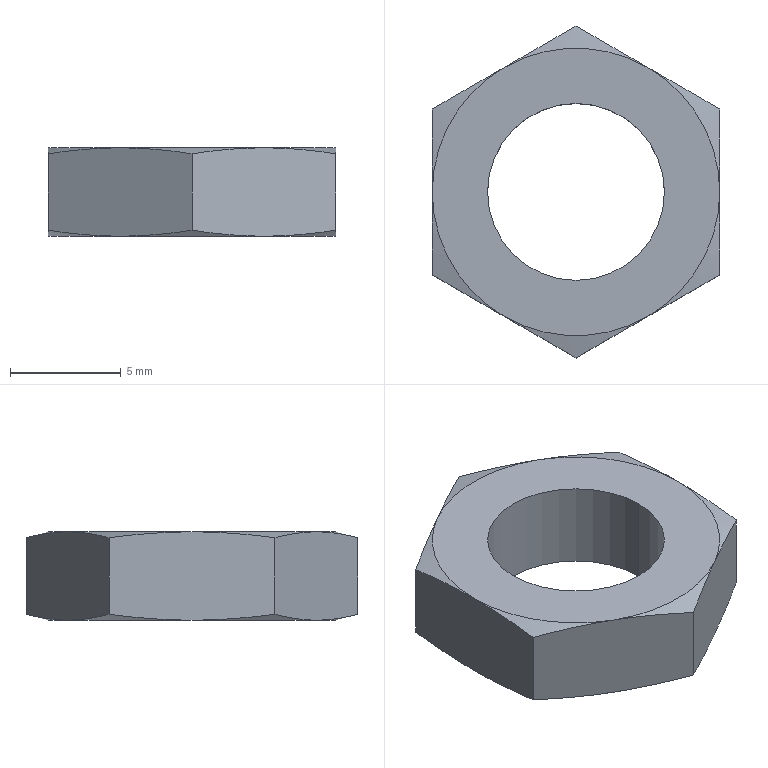Component | SolidWorks | GB_T6174-2000[HexThinNutNoChamferM8]-1 | 1 solid | 22 faces | box 13 x 15.01 x 4 mm | volume 382 mm3 | cone 12 | plane 8 | cylinder 2 | commonest cylinder face diameters 8 x2
build123d program:
from build123d import *

# Parameters (mm, degrees)
SKETCH1_R          = 4
BASE_EXTRUDE_DEPTH = 4
SKETCH2_OUTSIDE_W  = 106.414
SKETCH2_OUTSIDE_H  = 108.426
SKETCH2_OUTSIDE_R  = 6.5
CUT_EXTRUDE1_DEPTH = 11.704
CUT_EXTRUDE1_DRAFT = -75
SKETCH3_OUTSIDE_W  = 106.414
SKETCH3_OUTSIDE_H  = 108.426
SKETCH3_OUTSIDE_R  = 6.5
CUT_EXTRUDE2_DEPTH = 11.704
CUT_EXTRUDE2_DRAFT = -75


with BuildPart() as part:
    # Sketch1 → Base-Extrude (new body)
    with BuildSketch(Plane.XY):
        Polygon((0, 7.506), (-6.5, 3.753), (-6.5, -3.753), (0, -7.506), (6.5, -3.753), (6.5, 3.753), align=None)
        Circle(SKETCH1_R, mode=Mode.SUBTRACT)
    extrude(amount=BASE_EXTRUDE_DEPTH)


with BuildPart() as cut_extrude1_tool:
    # Sketch2 outside → Cut-Extrude1 (with draft: the straight prism first)
    with BuildSketch(Plane(origin=(0, 0, 0), x_dir=(-1, 0, 0), z_dir=(0, 0, -1))):
        Rectangle(SKETCH2_OUTSIDE_W, SKETCH2_OUTSIDE_H)
        Circle(SKETCH2_OUTSIDE_R, mode=Mode.SUBTRACT)
    extrude(amount=-CUT_EXTRUDE1_DEPTH)
    # Cut-Extrude1: the draft: its side faces are tilted about the plane it starts from
    cut_extrude1_sides = [cut_extrude1_tool.faces().sort_by_distance(p)[0] for p in [
        (0, -54.213, 5.852),
        (-53.207, 0, 5.852),
        (0, 54.213, 5.852),
        (53.207, 0, 5.852),
        (6.5, 0, 5.852),
    ]]
    draft(cut_extrude1_sides, Plane(origin=(0, 0, 0), x_dir=(-1, 0, 0), z_dir=(0, 0, -1)), CUT_EXTRUDE1_DRAFT)


with BuildPart() as part_1:
    add(part.part)

    # Cut-Extrude1: cut by cut_extrude1_tool
    add(cut_extrude1_tool.part, mode=Mode.SUBTRACT)


with BuildPart() as cut_extrude2_tool:
    # Sketch3 outside → Cut-Extrude2 (with draft: the straight prism first)
    with BuildSketch(Plane.XY.offset(4)):
        Rectangle(SKETCH3_OUTSIDE_W, SKETCH3_OUTSIDE_H)
        Circle(SKETCH3_OUTSIDE_R, mode=Mode.SUBTRACT)
    extrude(amount=-CUT_EXTRUDE2_DEPTH)
    # Cut-Extrude2: the draft: its side faces are tilted about the plane it starts from
    cut_extrude2_sides = [cut_extrude2_tool.faces().sort_by_distance(p)[0] for p in [
        (0, -54.213, -1.852),
        (53.207, 0, -1.852),
        (0, 54.213, -1.852),
        (-53.207, 0, -1.852),
        (-6.5, 0, -1.852),
    ]]
    draft(cut_extrude2_sides, Plane.XY.offset(4), CUT_EXTRUDE2_DRAFT)


with BuildPart() as part_2:
    add(part_1.part)

    # Cut-Extrude2: cut by cut_extrude2_tool
    add(cut_extrude2_tool.part, mode=Mode.SUBTRACT)


solid = part_2.part

# Placed as in the assembly
solid = solid.moved(Location((483.792, -540.614, 1168.971), (0, 0, 0)))
STEP:
#1=COLOUR_RGB('',0.7922,0.8196,0.9333);
#2=FILL_AREA_STYLE_COLOUR('',#1);
#3=FILL_AREA_STYLE('',(#2));
#4=SURFACE_STYLE_FILL_AREA(#3);
#5=SURFACE_SIDE_STYLE('',(#4));
#6=SURFACE_STYLE_USAGE(.BOTH.,#5);
#7=PRESENTATION_STYLE_ASSIGNMENT((#6));
#8=CARTESIAN_POINT('',(18.889,-21.284,46.18));
#9=VERTEX_POINT('',#8);
#10=CARTESIAN_POINT('',(19.204,-21.284,46.18));
#11=VERTEX_POINT('',#10);
#12=CARTESIAN_POINT('',(19.047,-21.284,46.18));
#13=DIRECTION('',(0.,0.,1.));
#14=DIRECTION('',(1.,0.,0.));
#15=AXIS2_PLACEMENT_3D('',#12,#13,#14);
#16=CIRCLE('',#15,0.1575);
#17=EDGE_CURVE('',#9,#11,#16,.T.);
#18=ORIENTED_EDGE('',*,*,#17,.T.);
#19=CARTESIAN_POINT('',(19.204,-21.284,46.022));
#20=VERTEX_POINT('',#19);
#21=CARTESIAN_POINT('',(19.204,-21.284,46.18));
#22=DIRECTION('',(0.,0.,-1.));
#23=VECTOR('',#22,39.37);
#24=LINE('',#21,#23);
#25=EDGE_CURVE('',#11,#20,#24,.T.);
#26=ORIENTED_EDGE('',*,*,#25,.T.);
#27=CARTESIAN_POINT('',(18.889,-21.284,46.022));
#28=VERTEX_POINT('',#27);
#29=CARTESIAN_POINT('',(19.047,-21.284,46.022));
#30=DIRECTION('',(0.,0.,1.));
#31=DIRECTION('',(1.,0.,0.));
#32=AXIS2_PLACEMENT_3D('',#29,#30,#31);
#33=CIRCLE('',#32,0.1575);
#34=EDGE_CURVE('',#28,#20,#33,.T.);
#35=ORIENTED_EDGE('',*,*,#34,.F.);
#36=CARTESIAN_POINT('',(18.889,-21.284,46.18));
#37=DIRECTION('',(0.,0.,-1.));
#38=VECTOR('',#37,39.37);
#39=LINE('',#36,#38);
#40=EDGE_CURVE('',#9,#28,#39,.T.);
#41=ORIENTED_EDGE('',*,*,#40,.F.);
#42=EDGE_LOOP('',(#18,#26,#35,#41));
#43=FACE_OUTER_BOUND('',#42,.T.);
#44=CARTESIAN_POINT('',(19.047,-21.284,46.18));
#45=DIRECTION('',(0.,0.,-1.));
#46=DIRECTION('',(-1.,0.,0.));
#47=AXIS2_PLACEMENT_3D('',#44,#45,#46);
#48=CYLINDRICAL_SURFACE('',#47,0.1575);
#49=ADVANCED_FACE('',(#43),#48,.F.);
#50=CARTESIAN_POINT('',(19.303,-21.136,46.169));
#51=VERTEX_POINT('',#50);
#52=CARTESIAN_POINT('',(19.175,-21.062,46.18));
#53=VERTEX_POINT('',#52);
#54=CARTESIAN_POINT('',(19.303,-21.136,46.169));
#55=CARTESIAN_POINT('',(19.26,-21.112,46.176));
#56=CARTESIAN_POINT('',(19.218,-21.087,46.18));
#57=CARTESIAN_POINT('',(19.175,-21.062,46.18));
#58=B_SPLINE_CURVE_WITH_KNOTS('',3,(#54,#55,#56,#57),.UNSPECIFIED.,.F.,.F.,(4,4),(0.00000023,0.003753),.UNSPECIFIED.);
#59=EDGE_CURVE('',#51,#53,#58,.T.);
#60=ORIENTED_EDGE('',*,*,#59,.F.);
#61=CARTESIAN_POINT('',(19.303,-21.136,46.033));
#62=VERTEX_POINT('',#61);
#63=CARTESIAN_POINT('',(19.303,-21.136,46.18));
#64=DIRECTION('',(0.,0.,-1.));
#65=VECTOR('',#64,39.37);
#66=LINE('',#63,#65);
#67=EDGE_CURVE('',#51,#62,#66,.T.);
#68=ORIENTED_EDGE('',*,*,#67,.T.);
#69=CARTESIAN_POINT('',(19.175,-21.062,46.022));
#70=VERTEX_POINT('',#69);
#71=CARTESIAN_POINT('',(19.175,-21.062,46.022));
#72=CARTESIAN_POINT('',(19.218,-21.087,46.022));
#73=CARTESIAN_POINT('',(19.26,-21.112,46.026));
#74=CARTESIAN_POINT('',(19.303,-21.136,46.033));
#75=B_SPLINE_CURVE_WITH_KNOTS('',3,(#71,#72,#73,#74),.UNSPECIFIED.,.F.,.F.,(4,4),(0.003753,0.007506),.UNSPECIFIED.);
#76=EDGE_CURVE('',#70,#62,#75,.T.);
#77=ORIENTED_EDGE('',*,*,#76,.F.);
#78=CARTESIAN_POINT('',(19.047,-20.989,46.033));
#79=VERTEX_POINT('',#78);
#80=CARTESIAN_POINT('',(19.047,-20.989,46.033));
#81=CARTESIAN_POINT('',(19.09,-21.013,46.026));
#82=CARTESIAN_POINT('',(19.132,-21.038,46.022));
#83=CARTESIAN_POINT('',(19.175,-21.062,46.022));
#84=B_SPLINE_CURVE_WITH_KNOTS('',3,(#80,#81,#82,#83),.UNSPECIFIED.,.F.,.F.,(4,4),(0.00000023,0.003753),.UNSPECIFIED.);
#85=EDGE_CURVE('',#79,#70,#84,.T.);
#86=ORIENTED_EDGE('',*,*,#85,.F.);
#87=CARTESIAN_POINT('',(19.047,-20.989,46.169));
#88=VERTEX_POINT('',#87);
#89=CARTESIAN_POINT('',(19.047,-20.989,46.18));
#90=DIRECTION('',(0.,0.,-1.));
#91=VECTOR('',#90,39.37);
#92=LINE('',#89,#91);
#93=EDGE_CURVE('',#88,#79,#92,.T.);
#94=ORIENTED_EDGE('',*,*,#93,.F.);
#95=CARTESIAN_POINT('',(19.175,-21.062,46.18));
#96=CARTESIAN_POINT('',(19.132,-21.038,46.18));
#97=CARTESIAN_POINT('',(19.09,-21.013,46.176));
#98=CARTESIAN_POINT('',(19.047,-20.989,46.169));
#99=B_SPLINE_CURVE_WITH_KNOTS('',3,(#95,#96,#97,#98),.UNSPECIFIED.,.F.,.F.,(4,4),(0.003753,0.007506),.UNSPECIFIED.);
#100=EDGE_CURVE('',#53,#88,#99,.T.);
#101=ORIENTED_EDGE('',*,*,#100,.F.);
#102=EDGE_LOOP('',(#60,#68,#77,#86,#94,#101));
#103=FACE_OUTER_BOUND('',#102,.T.);
#104=CARTESIAN_POINT('',(19.303,-21.136,46.18));
#105=DIRECTION('',(-0.5,-0.866,0.));
#106=DIRECTION('',(0.866,-0.5,0.));
#107=AXIS2_PLACEMENT_3D('',#104,#105,#106);
#108=PLANE('',#107);
#109=ADVANCED_FACE('',(#103),#108,.F.);
#110=CARTESIAN_POINT('',(18.919,-21.062,46.18));
#111=VERTEX_POINT('',#110);
#112=CARTESIAN_POINT('',(19.047,-20.989,46.169));
#113=CARTESIAN_POINT('',(19.004,-21.013,46.176));
#114=CARTESIAN_POINT('',(18.962,-21.038,46.18));
#115=CARTESIAN_POINT('',(18.919,-21.062,46.18));
#116=B_SPLINE_CURVE_WITH_KNOTS('',3,(#112,#113,#114,#115),.UNSPECIFIED.,.F.,.F.,(4,4),(0.00000023,0.003753),.UNSPECIFIED.);
#117=EDGE_CURVE('',#88,#111,#116,.T.);
#118=ORIENTED_EDGE('',*,*,#117,.F.);
#119=ORIENTED_EDGE('',*,*,#93,.T.);
#120=CARTESIAN_POINT('',(18.919,-21.062,46.022));
#121=VERTEX_POINT('',#120);
#122=CARTESIAN_POINT('',(18.919,-21.062,46.022));
#123=CARTESIAN_POINT('',(18.962,-21.038,46.022));
#124=CARTESIAN_POINT('',(19.004,-21.013,46.026));
#125=CARTESIAN_POINT('',(19.047,-20.989,46.033));
#126=B_SPLINE_CURVE_WITH_KNOTS('',3,(#122,#123,#124,#125),.UNSPECIFIED.,.F.,.F.,(4,4),(0.003753,0.007506),.UNSPECIFIED.);
#127=EDGE_CURVE('',#121,#79,#126,.T.);
#128=ORIENTED_EDGE('',*,*,#127,.F.);
#129=CARTESIAN_POINT('',(18.791,-21.136,46.033));
#130=VERTEX_POINT('',#129);
#131=CARTESIAN_POINT('',(18.791,-21.136,46.033));
#132=CARTESIAN_POINT('',(18.834,-21.112,46.026));
#133=CARTESIAN_POINT('',(18.876,-21.087,46.022));
#134=CARTESIAN_POINT('',(18.919,-21.062,46.022));
#135=B_SPLINE_CURVE_WITH_KNOTS('',3,(#131,#132,#133,#134),.UNSPECIFIED.,.F.,.F.,(4,4),(0.00000023,0.003753),.UNSPECIFIED.);
#136=EDGE_CURVE('',#130,#121,#135,.T.);
#137=ORIENTED_EDGE('',*,*,#136,.F.);
#138=CARTESIAN_POINT('',(18.791,-21.136,46.169));
#139=VERTEX_POINT('',#138);
#140=CARTESIAN_POINT('',(18.791,-21.136,46.18));
#141=DIRECTION('',(0.,0.,-1.));
#142=VECTOR('',#141,39.37);
#143=LINE('',#140,#142);
#144=EDGE_CURVE('',#139,#130,#143,.T.);
#145=ORIENTED_EDGE('',*,*,#144,.F.);
#146=CARTESIAN_POINT('',(18.919,-21.062,46.18));
#147=CARTESIAN_POINT('',(18.876,-21.087,46.18));
#148=CARTESIAN_POINT('',(18.834,-21.112,46.176));
#149=CARTESIAN_POINT('',(18.791,-21.136,46.169));
#150=B_SPLINE_CURVE_WITH_KNOTS('',3,(#146,#147,#148,#149),.UNSPECIFIED.,.F.,.F.,(4,4),(0.003753,0.007506),.UNSPECIFIED.);
#151=EDGE_CURVE('',#111,#139,#150,.T.);
#152=ORIENTED_EDGE('',*,*,#151,.F.);
#153=EDGE_LOOP('',(#118,#119,#128,#137,#145,#152));
#154=FACE_OUTER_BOUND('',#153,.T.);
#155=CARTESIAN_POINT('',(19.047,-20.989,46.18));
#156=DIRECTION('',(0.5,-0.866,0.));
#157=DIRECTION('',(0.866,0.5,0.));
#158=AXIS2_PLACEMENT_3D('',#155,#156,#157);
#159=PLANE('',#158);
#160=ADVANCED_FACE('',(#154),#159,.F.);
#161=CARTESIAN_POINT('',(18.791,-21.284,46.18));
#162=VERTEX_POINT('',#161);
#163=CARTESIAN_POINT('',(18.791,-21.136,46.169));
#164=CARTESIAN_POINT('',(18.791,-21.185,46.176));
#165=CARTESIAN_POINT('',(18.791,-21.235,46.18));
#166=CARTESIAN_POINT('',(18.791,-21.284,46.18));
#167=B_SPLINE_CURVE_WITH_KNOTS('',3,(#163,#164,#165,#166),.UNSPECIFIED.,.F.,.F.,(4,4),(0.01751,0.02129),.UNSPECIFIED.);
#168=EDGE_CURVE('',#139,#162,#167,.T.);
#169=ORIENTED_EDGE('',*,*,#168,.F.);
#170=ORIENTED_EDGE('',*,*,#144,.T.);
#171=CARTESIAN_POINT('',(18.791,-21.284,46.022));
#172=VERTEX_POINT('',#171);
#173=CARTESIAN_POINT('',(18.791,-21.284,46.022));
#174=CARTESIAN_POINT('',(18.791,-21.235,46.022));
#175=CARTESIAN_POINT('',(18.791,-21.185,46.027));
#176=CARTESIAN_POINT('',(18.791,-21.136,46.033));
#177=B_SPLINE_CURVE_WITH_KNOTS('',3,(#173,#174,#175,#176),.UNSPECIFIED.,.F.,.F.,(4,4),(0.01018,0.01396),.UNSPECIFIED.);
#178=EDGE_CURVE('',#172,#130,#177,.T.);
#179=ORIENTED_EDGE('',*,*,#178,.F.);
#180=CARTESIAN_POINT('',(18.791,-21.432,46.033));
#181=VERTEX_POINT('',#180);
#182=CARTESIAN_POINT('',(18.791,-21.432,46.033));
#183=CARTESIAN_POINT('',(18.791,-21.407,46.03));
#184=CARTESIAN_POINT('',(18.791,-21.383,46.027));
#185=CARTESIAN_POINT('',(18.791,-21.333,46.023));
#186=CARTESIAN_POINT('',(18.791,-21.309,46.022));
#187=CARTESIAN_POINT('',(18.791,-21.284,46.022));
#188=B_SPLINE_CURVE_WITH_KNOTS('',3,(#182,#183,#184,#185,#186,#187),.UNSPECIFIED.,.F.,.F.,(4,2,4),(0.006406,0.008292,0.01018),.UNSPECIFIED.);
#189=EDGE_CURVE('',#181,#172,#188,.T.);
#190=ORIENTED_EDGE('',*,*,#189,.F.);
#191=CARTESIAN_POINT('',(18.791,-21.432,46.169));
#192=VERTEX_POINT('',#191);
#193=CARTESIAN_POINT('',(18.791,-21.432,46.18));
#194=DIRECTION('',(0.,0.,-1.));
#195=VECTOR('',#194,39.37);
#196=LINE('',#193,#195);
#197=EDGE_CURVE('',#192,#181,#196,.T.);
#198=ORIENTED_EDGE('',*,*,#197,.F.);
#199=CARTESIAN_POINT('',(18.791,-21.284,46.18));
#200=CARTESIAN_POINT('',(18.791,-21.309,46.18));
#201=CARTESIAN_POINT('',(18.791,-21.333,46.179));
#202=CARTESIAN_POINT('',(18.791,-21.383,46.175));
#203=CARTESIAN_POINT('',(18.791,-21.407,46.173));
#204=CARTESIAN_POINT('',(18.791,-21.432,46.169));
#205=B_SPLINE_CURVE_WITH_KNOTS('',3,(#199,#200,#201,#202,#203,#204),.UNSPECIFIED.,.F.,.F.,(4,2,4),(0.02129,0.02317,0.02505),.UNSPECIFIED.);
#206=EDGE_CURVE('',#162,#192,#205,.T.);
#207=ORIENTED_EDGE('',*,*,#206,.F.);
#208=EDGE_LOOP('',(#169,#170,#179,#190,#198,#207));
#209=FACE_OUTER_BOUND('',#208,.T.);
#210=CARTESIAN_POINT('',(18.791,-21.136,46.18));
#211=DIRECTION('',(1.,0.,0.));
#212=DIRECTION('',(0.,0.,-1.));
#213=AXIS2_PLACEMENT_3D('',#210,#211,#212);
#214=PLANE('',#213);
#215=ADVANCED_FACE('',(#209),#214,.F.);
#216=CARTESIAN_POINT('',(18.919,-21.506,46.18));
#217=VERTEX_POINT('',#216);
#218=CARTESIAN_POINT('',(18.791,-21.432,46.169));
#219=CARTESIAN_POINT('',(18.834,-21.456,46.176));
#220=CARTESIAN_POINT('',(18.876,-21.481,46.18));
#221=CARTESIAN_POINT('',(18.919,-21.506,46.18));
#222=B_SPLINE_CURVE_WITH_KNOTS('',3,(#218,#219,#220,#221),.UNSPECIFIED.,.F.,.F.,(4,4),(0.00000023,0.003753),.UNSPECIFIED.);
#223=EDGE_CURVE('',#192,#217,#222,.T.);
#224=ORIENTED_EDGE('',*,*,#223,.F.);
#225=ORIENTED_EDGE('',*,*,#197,.T.);
#226=CARTESIAN_POINT('',(18.919,-21.506,46.022));
#227=VERTEX_POINT('',#226);
#228=CARTESIAN_POINT('',(18.919,-21.506,46.022));
#229=CARTESIAN_POINT('',(18.876,-21.481,46.022));
#230=CARTESIAN_POINT('',(18.834,-21.456,46.026));
#231=CARTESIAN_POINT('',(18.791,-21.432,46.033));
#232=B_SPLINE_CURVE_WITH_KNOTS('',3,(#228,#229,#230,#231),.UNSPECIFIED.,.F.,.F.,(4,4),(0.003753,0.007506),.UNSPECIFIED.);
#233=EDGE_CURVE('',#227,#181,#232,.T.);
#234=ORIENTED_EDGE('',*,*,#233,.F.);
#235=CARTESIAN_POINT('',(19.047,-21.58,46.033));
#236=VERTEX_POINT('',#235);
#237=CARTESIAN_POINT('',(19.047,-21.58,46.033));
#238=CARTESIAN_POINT('',(19.004,-21.555,46.026));
#239=CARTESIAN_POINT('',(18.962,-21.53,46.022));
#240=CARTESIAN_POINT('',(18.919,-21.506,46.022));
#241=B_SPLINE_CURVE_WITH_KNOTS('',3,(#237,#238,#239,#240),.UNSPECIFIED.,.F.,.F.,(4,4),(0.00000023,0.003753),.UNSPECIFIED.);
#242=EDGE_CURVE('',#236,#227,#241,.T.);
#243=ORIENTED_EDGE('',*,*,#242,.F.);
#244=CARTESIAN_POINT('',(19.047,-21.58,46.169));
#245=VERTEX_POINT('',#244);
#246=CARTESIAN_POINT('',(19.047,-21.58,46.18));
#247=DIRECTION('',(0.,0.,-1.));
#248=VECTOR('',#247,39.37);
#249=LINE('',#246,#248);
#250=EDGE_CURVE('',#245,#236,#249,.T.);
#251=ORIENTED_EDGE('',*,*,#250,.F.);
#252=CARTESIAN_POINT('',(18.919,-21.506,46.18));
#253=CARTESIAN_POINT('',(18.962,-21.53,46.18));
#254=CARTESIAN_POINT('',(19.004,-21.555,46.176));
#255=CARTESIAN_POINT('',(19.047,-21.58,46.169));
#256=B_SPLINE_CURVE_WITH_KNOTS('',3,(#252,#253,#254,#255),.UNSPECIFIED.,.F.,.F.,(4,4),(0.003753,0.007506),.UNSPECIFIED.);
#257=EDGE_CURVE('',#217,#245,#256,.T.);
#258=ORIENTED_EDGE('',*,*,#257,.F.);
#259=EDGE_LOOP('',(#224,#225,#234,#243,#251,#258));
#260=FACE_OUTER_BOUND('',#259,.T.);
#261=CARTESIAN_POINT('',(18.791,-21.432,46.18));
#262=DIRECTION('',(0.5,0.866,0.));
#263=DIRECTION('',(-0.866,0.5,0.));
#264=AXIS2_PLACEMENT_3D('',#261,#262,#263);
#265=PLANE('',#264);
#266=ADVANCED_FACE('',(#260),#265,.F.);
#267=CARTESIAN_POINT('',(19.175,-21.506,46.18));
#268=VERTEX_POINT('',#267);
#269=CARTESIAN_POINT('',(19.047,-21.58,46.169));
#270=CARTESIAN_POINT('',(19.09,-21.555,46.176));
#271=CARTESIAN_POINT('',(19.132,-21.53,46.18));
#272=CARTESIAN_POINT('',(19.175,-21.506,46.18));
#273=B_SPLINE_CURVE_WITH_KNOTS('',3,(#269,#270,#271,#272),.UNSPECIFIED.,.F.,.F.,(4,4),(0.00000023,0.003753),.UNSPECIFIED.);
#274=EDGE_CURVE('',#245,#268,#273,.T.);
#275=ORIENTED_EDGE('',*,*,#274,.F.);
#276=ORIENTED_EDGE('',*,*,#250,.T.);
#277=CARTESIAN_POINT('',(19.175,-21.506,46.022));
#278=VERTEX_POINT('',#277);
#279=CARTESIAN_POINT('',(19.175,-21.506,46.022));
#280=CARTESIAN_POINT('',(19.132,-21.53,46.022));
#281=CARTESIAN_POINT('',(19.09,-21.555,46.026));
#282=CARTESIAN_POINT('',(19.047,-21.58,46.033));
#283=B_SPLINE_CURVE_WITH_KNOTS('',3,(#279,#280,#281,#282),.UNSPECIFIED.,.F.,.F.,(4,4),(0.003753,0.007506),.UNSPECIFIED.);
#284=EDGE_CURVE('',#278,#236,#283,.T.);
#285=ORIENTED_EDGE('',*,*,#284,.F.);
#286=CARTESIAN_POINT('',(19.303,-21.432,46.033));
#287=VERTEX_POINT('',#286);
#288=CARTESIAN_POINT('',(19.303,-21.432,46.033));
#289=CARTESIAN_POINT('',(19.26,-21.456,46.026));
#290=CARTESIAN_POINT('',(19.218,-21.481,46.022));
#291=CARTESIAN_POINT('',(19.175,-21.506,46.022));
#292=B_SPLINE_CURVE_WITH_KNOTS('',3,(#288,#289,#290,#291),.UNSPECIFIED.,.F.,.F.,(4,4),(0.00000023,0.003753),.UNSPECIFIED.);
#293=EDGE_CURVE('',#287,#278,#292,.T.);
#294=ORIENTED_EDGE('',*,*,#293,.F.);
#295=CARTESIAN_POINT('',(19.303,-21.432,46.169));
#296=VERTEX_POINT('',#295);
#297=CARTESIAN_POINT('',(19.303,-21.432,46.18));
#298=DIRECTION('',(0.,0.,-1.));
#299=VECTOR('',#298,39.37);
#300=LINE('',#297,#299);
#301=EDGE_CURVE('',#296,#287,#300,.T.);
#302=ORIENTED_EDGE('',*,*,#301,.F.);
#303=CARTESIAN_POINT('',(19.175,-21.506,46.18));
#304=CARTESIAN_POINT('',(19.218,-21.481,46.18));
#305=CARTESIAN_POINT('',(19.26,-21.456,46.176));
#306=CARTESIAN_POINT('',(19.303,-21.432,46.169));
#307=B_SPLINE_CURVE_WITH_KNOTS('',3,(#303,#304,#305,#306),.UNSPECIFIED.,.F.,.F.,(4,4),(0.003753,0.007506),.UNSPECIFIED.);
#308=EDGE_CURVE('',#268,#296,#307,.T.);
#309=ORIENTED_EDGE('',*,*,#308,.F.);
#310=EDGE_LOOP('',(#275,#276,#285,#294,#302,#309));
#311=FACE_OUTER_BOUND('',#310,.T.);
#312=CARTESIAN_POINT('',(19.047,-21.58,46.18));
#313=DIRECTION('',(-0.5,0.866,0.));
#314=DIRECTION('',(-0.866,-0.5,0.));
#315=AXIS2_PLACEMENT_3D('',#312,#313,#314);
#316=PLANE('',#315);
#317=ADVANCED_FACE('',(#311),#316,.F.);
#318=CARTESIAN_POINT('',(19.303,-21.284,46.18));
#319=VERTEX_POINT('',#318);
#320=CARTESIAN_POINT('',(19.303,-21.432,46.169));
#321=CARTESIAN_POINT('',(19.303,-21.407,46.173));
#322=CARTESIAN_POINT('',(19.303,-21.383,46.175));
#323=CARTESIAN_POINT('',(19.303,-21.333,46.179));
#324=CARTESIAN_POINT('',(19.303,-21.309,46.18));
#325=CARTESIAN_POINT('',(19.303,-21.284,46.18));
#326=B_SPLINE_CURVE_WITH_KNOTS('',3,(#320,#321,#322,#323,#324,#325),.UNSPECIFIED.,.F.,.F.,(4,2,4),(0.006406,0.008292,0.01018),.UNSPECIFIED.);
#327=EDGE_CURVE('',#296,#319,#326,.T.);
#328=ORIENTED_EDGE('',*,*,#327,.F.);
#329=ORIENTED_EDGE('',*,*,#301,.T.);
#330=CARTESIAN_POINT('',(19.303,-21.284,46.022));
#331=VERTEX_POINT('',#330);
#332=CARTESIAN_POINT('',(19.303,-21.284,46.022));
#333=CARTESIAN_POINT('',(19.303,-21.309,46.022));
#334=CARTESIAN_POINT('',(19.303,-21.333,46.023));
#335=CARTESIAN_POINT('',(19.303,-21.383,46.027));
#336=CARTESIAN_POINT('',(19.303,-21.407,46.03));
#337=CARTESIAN_POINT('',(19.303,-21.432,46.033));
#338=B_SPLINE_CURVE_WITH_KNOTS('',3,(#332,#333,#334,#335,#336,#337),.UNSPECIFIED.,.F.,.F.,(4,2,4),(0.02129,0.02317,0.02505),.UNSPECIFIED.);
#339=EDGE_CURVE('',#331,#287,#338,.T.);
#340=ORIENTED_EDGE('',*,*,#339,.F.);
#341=CARTESIAN_POINT('',(19.303,-21.136,46.033));
#342=CARTESIAN_POINT('',(19.303,-21.185,46.027));
#343=CARTESIAN_POINT('',(19.303,-21.235,46.022));
#344=CARTESIAN_POINT('',(19.303,-21.284,46.022));
#345=B_SPLINE_CURVE_WITH_KNOTS('',3,(#341,#342,#343,#344),.UNSPECIFIED.,.F.,.F.,(4,4),(0.01751,0.02129),.UNSPECIFIED.);
#346=EDGE_CURVE('',#62,#331,#345,.T.);
#347=ORIENTED_EDGE('',*,*,#346,.F.);
#348=ORIENTED_EDGE('',*,*,#67,.F.);
#349=CARTESIAN_POINT('',(19.303,-21.284,46.18));
#350=CARTESIAN_POINT('',(19.303,-21.235,46.18));
#351=CARTESIAN_POINT('',(19.303,-21.185,46.176));
#352=CARTESIAN_POINT('',(19.303,-21.136,46.169));
#353=B_SPLINE_CURVE_WITH_KNOTS('',3,(#349,#350,#351,#352),.UNSPECIFIED.,.F.,.F.,(4,4),(0.01018,0.01396),.UNSPECIFIED.);
#354=EDGE_CURVE('',#319,#51,#353,.T.);
#355=ORIENTED_EDGE('',*,*,#354,.F.);
#356=EDGE_LOOP('',(#328,#329,#340,#347,#348,#355));
#357=FACE_OUTER_BOUND('',#356,.T.);
#358=CARTESIAN_POINT('',(19.303,-21.432,46.18));
#359=DIRECTION('',(-1.,0.,0.));
#360=DIRECTION('',(0.,0.,1.));
#361=AXIS2_PLACEMENT_3D('',#358,#359,#360);
#362=PLANE('',#361);
#363=ADVANCED_FACE('',(#357),#362,.F.);
#364=ORIENTED_EDGE('',*,*,#17,.F.);
#365=CARTESIAN_POINT('',(19.047,-21.284,46.18));
#366=DIRECTION('',(0.,0.,1.));
#367=DIRECTION('',(1.,0.,0.));
#368=AXIS2_PLACEMENT_3D('',#365,#366,#367);
#369=CIRCLE('',#368,0.1575);
#370=EDGE_CURVE('',#11,#9,#369,.T.);
#371=ORIENTED_EDGE('',*,*,#370,.F.);
#372=EDGE_LOOP('',(#364,#371));
#373=FACE_BOUND('',#372,.T.);
#374=CARTESIAN_POINT('',(19.047,-21.284,46.18));
#375=DIRECTION('',(0.,0.,1.));
#376=DIRECTION('',(1.,0.,0.));
#377=AXIS2_PLACEMENT_3D('',#374,#375,#376);
#378=CIRCLE('',#377,0.2559);
#379=EDGE_CURVE('',#268,#319,#378,.T.);
#380=ORIENTED_EDGE('',*,*,#379,.T.);
#381=CARTESIAN_POINT('',(19.047,-21.284,46.18));
#382=DIRECTION('',(0.,0.,1.));
#383=DIRECTION('',(1.,0.,0.));
#384=AXIS2_PLACEMENT_3D('',#381,#382,#383);
#385=CIRCLE('',#384,0.2559);
#386=EDGE_CURVE('',#319,#53,#385,.T.);
#387=ORIENTED_EDGE('',*,*,#386,.T.);
#388=CARTESIAN_POINT('',(19.047,-21.284,46.18));
#389=DIRECTION('',(0.,0.,1.));
#390=DIRECTION('',(1.,0.,0.));
#391=AXIS2_PLACEMENT_3D('',#388,#389,#390);
#392=CIRCLE('',#391,0.2559);
#393=EDGE_CURVE('',#53,#111,#392,.T.);
#394=ORIENTED_EDGE('',*,*,#393,.T.);
#395=CARTESIAN_POINT('',(19.047,-21.284,46.18));
#396=DIRECTION('',(0.,0.,1.));
#397=DIRECTION('',(1.,0.,0.));
#398=AXIS2_PLACEMENT_3D('',#395,#396,#397);
#399=CIRCLE('',#398,0.2559);
#400=EDGE_CURVE('',#111,#162,#399,.T.);
#401=ORIENTED_EDGE('',*,*,#400,.T.);
#402=CARTESIAN_POINT('',(19.047,-21.284,46.18));
#403=DIRECTION('',(0.,0.,1.));
#404=DIRECTION('',(1.,0.,0.));
#405=AXIS2_PLACEMENT_3D('',#402,#403,#404);
#406=CIRCLE('',#405,0.2559);
#407=EDGE_CURVE('',#162,#217,#406,.T.);
#408=ORIENTED_EDGE('',*,*,#407,.T.);
#409=CARTESIAN_POINT('',(19.047,-21.284,46.18));
#410=DIRECTION('',(0.,0.,1.));
#411=DIRECTION('',(1.,0.,0.));
#412=AXIS2_PLACEMENT_3D('',#409,#410,#411);
#413=CIRCLE('',#412,0.2559);
#414=EDGE_CURVE('',#217,#268,#413,.T.);
#415=ORIENTED_EDGE('',*,*,#414,.T.);
#416=EDGE_LOOP('',(#380,#387,#394,#401,#408,#415));
#417=FACE_OUTER_BOUND('',#416,.T.);
#418=CARTESIAN_POINT('',(18.791,-20.841,46.18));
#419=DIRECTION('',(0.,0.,1.));
#420=DIRECTION('',(1.,0.,0.));
#421=AXIS2_PLACEMENT_3D('',#418,#419,#420);
#422=PLANE('',#421);
#423=ADVANCED_FACE('',(#373,#417),#422,.T.);
#424=ORIENTED_EDGE('',*,*,#34,.T.);
#425=CARTESIAN_POINT('',(19.047,-21.284,46.022));
#426=DIRECTION('',(0.,0.,1.));
#427=DIRECTION('',(1.,0.,0.));
#428=AXIS2_PLACEMENT_3D('',#425,#426,#427);
#429=CIRCLE('',#428,0.1575);
#430=EDGE_CURVE('',#20,#28,#429,.T.);
#431=ORIENTED_EDGE('',*,*,#430,.T.);
#432=EDGE_LOOP('',(#424,#431));
#433=FACE_BOUND('',#432,.T.);
#434=CARTESIAN_POINT('',(19.047,-21.284,46.022));
#435=DIRECTION('',(0.,0.,-1.));
#436=DIRECTION('',(-1.,0.,0.));
#437=AXIS2_PLACEMENT_3D('',#434,#435,#436);
#438=CIRCLE('',#437,0.2559);
#439=EDGE_CURVE('',#70,#331,#438,.T.);
#440=ORIENTED_EDGE('',*,*,#439,.T.);
#441=CARTESIAN_POINT('',(19.047,-21.284,46.022));
#442=DIRECTION('',(0.,0.,-1.));
#443=DIRECTION('',(-1.,0.,0.));
#444=AXIS2_PLACEMENT_3D('',#441,#442,#443);
#445=CIRCLE('',#444,0.2559);
#446=EDGE_CURVE('',#331,#278,#445,.T.);
#447=ORIENTED_EDGE('',*,*,#446,.T.);
#448=CARTESIAN_POINT('',(19.047,-21.284,46.022));
#449=DIRECTION('',(0.,0.,-1.));
#450=DIRECTION('',(-1.,0.,0.));
#451=AXIS2_PLACEMENT_3D('',#448,#449,#450);
#452=CIRCLE('',#451,0.2559);
#453=EDGE_CURVE('',#278,#227,#452,.T.);
#454=ORIENTED_EDGE('',*,*,#453,.T.);
#455=CARTESIAN_POINT('',(19.047,-21.284,46.022));
#456=DIRECTION('',(0.,0.,-1.));
#457=DIRECTION('',(-1.,0.,0.));
#458=AXIS2_PLACEMENT_3D('',#455,#456,#457);
#459=CIRCLE('',#458,0.2559);
#460=EDGE_CURVE('',#227,#172,#459,.T.);
#461=ORIENTED_EDGE('',*,*,#460,.T.);
#462=CARTESIAN_POINT('',(19.047,-21.284,46.022));
#463=DIRECTION('',(0.,0.,-1.));
#464=DIRECTION('',(-1.,0.,0.));
#465=AXIS2_PLACEMENT_3D('',#462,#463,#464);
#466=CIRCLE('',#465,0.2559);
#467=EDGE_CURVE('',#172,#121,#466,.T.);
#468=ORIENTED_EDGE('',*,*,#467,.T.);
#469=CARTESIAN_POINT('',(19.047,-21.284,46.022));
#470=DIRECTION('',(0.,0.,-1.));
#471=DIRECTION('',(-1.,0.,0.));
#472=AXIS2_PLACEMENT_3D('',#469,#470,#471);
#473=CIRCLE('',#472,0.2559);
#474=EDGE_CURVE('',#121,#70,#473,.T.);
#475=ORIENTED_EDGE('',*,*,#474,.T.);
#476=EDGE_LOOP('',(#440,#447,#454,#461,#468,#475));
#477=FACE_OUTER_BOUND('',#476,.T.);
#478=CARTESIAN_POINT('',(18.791,-20.841,46.022));
#479=DIRECTION('',(0.,0.,1.));
#480=DIRECTION('',(1.,0.,0.));
#481=AXIS2_PLACEMENT_3D('',#478,#479,#480);
#482=PLANE('',#481);
#483=ADVANCED_FACE('',(#433,#477),#482,.F.);
#484=ORIENTED_EDGE('',*,*,#25,.F.);
#485=ORIENTED_EDGE('',*,*,#370,.T.);
#486=ORIENTED_EDGE('',*,*,#40,.T.);
#487=ORIENTED_EDGE('',*,*,#430,.F.);
#488=EDGE_LOOP('',(#484,#485,#486,#487));
#489=FACE_OUTER_BOUND('',#488,.T.);
#490=CARTESIAN_POINT('',(19.047,-21.284,46.18));
#491=DIRECTION('',(0.,0.,-1.));
#492=DIRECTION('',(-1.,0.,0.));
#493=AXIS2_PLACEMENT_3D('',#490,#491,#492);
#494=CYLINDRICAL_SURFACE('',#493,0.1575);
#495=ADVANCED_FACE('',(#489),#494,.F.);
#496=ORIENTED_EDGE('',*,*,#293,.T.);
#497=ORIENTED_EDGE('',*,*,#446,.F.);
#498=ORIENTED_EDGE('',*,*,#339,.T.);
#499=EDGE_LOOP('',(#496,#497,#498));
#500=FACE_OUTER_BOUND('',#499,.T.);
#501=CARTESIAN_POINT('',(19.047,-21.284,46.022));
#502=DIRECTION('',(0.,0.,1.));
#503=DIRECTION('',(-1.,0.,0.));
#504=AXIS2_PLACEMENT_3D('',#501,#502,#503);
#505=CONICAL_SURFACE('',#504,0.2559,1.309);
#506=ADVANCED_FACE('',(#500),#505,.T.);
#507=ORIENTED_EDGE('',*,*,#76,.T.);
#508=ORIENTED_EDGE('',*,*,#346,.T.);
#509=ORIENTED_EDGE('',*,*,#439,.F.);
#510=EDGE_LOOP('',(#507,#508,#509));
#511=FACE_OUTER_BOUND('',#510,.T.);
#512=CARTESIAN_POINT('',(19.047,-21.284,46.022));
#513=DIRECTION('',(0.,0.,1.));
#514=DIRECTION('',(-1.,0.,0.));
#515=AXIS2_PLACEMENT_3D('',#512,#513,#514);
#516=CONICAL_SURFACE('',#515,0.2559,1.309);
#517=ADVANCED_FACE('',(#511),#516,.T.);
#518=ORIENTED_EDGE('',*,*,#242,.T.);
#519=ORIENTED_EDGE('',*,*,#453,.F.);
#520=ORIENTED_EDGE('',*,*,#284,.T.);
#521=EDGE_LOOP('',(#518,#519,#520));
#522=FACE_OUTER_BOUND('',#521,.T.);
#523=CARTESIAN_POINT('',(19.047,-21.284,46.022));
#524=DIRECTION('',(0.,0.,1.));
#525=DIRECTION('',(-1.,0.,0.));
#526=AXIS2_PLACEMENT_3D('',#523,#524,#525);
#527=CONICAL_SURFACE('',#526,0.2559,1.309);
#528=ADVANCED_FACE('',(#522),#527,.T.);
#529=ORIENTED_EDGE('',*,*,#189,.T.);
#530=ORIENTED_EDGE('',*,*,#460,.F.);
#531=ORIENTED_EDGE('',*,*,#233,.T.);
#532=EDGE_LOOP('',(#529,#530,#531));
#533=FACE_OUTER_BOUND('',#532,.T.);
#534=CARTESIAN_POINT('',(19.047,-21.284,46.022));
#535=DIRECTION('',(0.,0.,1.));
#536=DIRECTION('',(-1.,0.,0.));
#537=AXIS2_PLACEMENT_3D('',#534,#535,#536);
#538=CONICAL_SURFACE('',#537,0.2559,1.309);
#539=ADVANCED_FACE('',(#533),#538,.T.);
#540=ORIENTED_EDGE('',*,*,#178,.T.);
#541=ORIENTED_EDGE('',*,*,#136,.T.);
#542=ORIENTED_EDGE('',*,*,#467,.F.);
#543=EDGE_LOOP('',(#540,#541,#542));
#544=FACE_OUTER_BOUND('',#543,.T.);
#545=CARTESIAN_POINT('',(19.047,-21.284,46.022));
#546=DIRECTION('',(0.,0.,1.));
#547=DIRECTION('',(-1.,0.,0.));
#548=AXIS2_PLACEMENT_3D('',#545,#546,#547);
#549=CONICAL_SURFACE('',#548,0.2559,1.309);
#550=ADVANCED_FACE('',(#544),#549,.T.);
#551=ORIENTED_EDGE('',*,*,#127,.T.);
#552=ORIENTED_EDGE('',*,*,#85,.T.);
#553=ORIENTED_EDGE('',*,*,#474,.F.);
#554=EDGE_LOOP('',(#551,#552,#553));
#555=FACE_OUTER_BOUND('',#554,.T.);
#556=CARTESIAN_POINT('',(19.047,-21.284,46.022));
#557=DIRECTION('',(0.,0.,1.));
#558=DIRECTION('',(-1.,0.,0.));
#559=AXIS2_PLACEMENT_3D('',#556,#557,#558);
#560=CONICAL_SURFACE('',#559,0.2559,1.309);
#561=ADVANCED_FACE('',(#555),#560,.T.);
#562=ORIENTED_EDGE('',*,*,#308,.T.);
#563=ORIENTED_EDGE('',*,*,#327,.T.);
#564=ORIENTED_EDGE('',*,*,#379,.F.);
#565=EDGE_LOOP('',(#562,#563,#564));
#566=FACE_OUTER_BOUND('',#565,.T.);
#567=CARTESIAN_POINT('',(19.047,-21.284,46.18));
#568=DIRECTION('',(0.,0.,-1.));
#569=DIRECTION('',(1.,0.,0.));
#570=AXIS2_PLACEMENT_3D('',#567,#568,#569);
#571=CONICAL_SURFACE('',#570,0.2559,1.309);
#572=ADVANCED_FACE('',(#566),#571,.T.);
#573=ORIENTED_EDGE('',*,*,#257,.T.);
#574=ORIENTED_EDGE('',*,*,#274,.T.);
#575=ORIENTED_EDGE('',*,*,#414,.F.);
#576=EDGE_LOOP('',(#573,#574,#575));
#577=FACE_OUTER_BOUND('',#576,.T.);
#578=CARTESIAN_POINT('',(19.047,-21.284,46.18));
#579=DIRECTION('',(0.,0.,-1.));
#580=DIRECTION('',(1.,0.,0.));
#581=AXIS2_PLACEMENT_3D('',#578,#579,#580);
#582=CONICAL_SURFACE('',#581,0.2559,1.309);
#583=ADVANCED_FACE('',(#577),#582,.T.);
#584=ORIENTED_EDGE('',*,*,#206,.T.);
#585=ORIENTED_EDGE('',*,*,#223,.T.);
#586=ORIENTED_EDGE('',*,*,#407,.F.);
#587=EDGE_LOOP('',(#584,#585,#586));
#588=FACE_OUTER_BOUND('',#587,.T.);
#589=CARTESIAN_POINT('',(19.047,-21.284,46.18));
#590=DIRECTION('',(0.,0.,-1.));
#591=DIRECTION('',(1.,0.,0.));
#592=AXIS2_PLACEMENT_3D('',#589,#590,#591);
#593=CONICAL_SURFACE('',#592,0.2559,1.309);
#594=ADVANCED_FACE('',(#588),#593,.T.);
#595=ORIENTED_EDGE('',*,*,#151,.T.);
#596=ORIENTED_EDGE('',*,*,#168,.T.);
#597=ORIENTED_EDGE('',*,*,#400,.F.);
#598=EDGE_LOOP('',(#595,#596,#597));
#599=FACE_OUTER_BOUND('',#598,.T.);
#600=CARTESIAN_POINT('',(19.047,-21.284,46.18));
#601=DIRECTION('',(0.,0.,-1.));
#602=DIRECTION('',(1.,0.,0.));
#603=AXIS2_PLACEMENT_3D('',#600,#601,#602);
#604=CONICAL_SURFACE('',#603,0.2559,1.309);
#605=ADVANCED_FACE('',(#599),#604,.T.);
#606=ORIENTED_EDGE('',*,*,#100,.T.);
#607=ORIENTED_EDGE('',*,*,#117,.T.);
#608=ORIENTED_EDGE('',*,*,#393,.F.);
#609=EDGE_LOOP('',(#606,#607,#608));
#610=FACE_OUTER_BOUND('',#609,.T.);
#611=CARTESIAN_POINT('',(19.047,-21.284,46.18));
#612=DIRECTION('',(0.,0.,-1.));
#613=DIRECTION('',(1.,0.,0.));
#614=AXIS2_PLACEMENT_3D('',#611,#612,#613);
#615=CONICAL_SURFACE('',#614,0.2559,1.309);
#616=ADVANCED_FACE('',(#610),#615,.T.);
#617=ORIENTED_EDGE('',*,*,#59,.T.);
#618=ORIENTED_EDGE('',*,*,#386,.F.);
#619=ORIENTED_EDGE('',*,*,#354,.T.);
#620=EDGE_LOOP('',(#617,#618,#619));
#621=FACE_OUTER_BOUND('',#620,.T.);
#622=CARTESIAN_POINT('',(19.047,-21.284,46.18));
#623=DIRECTION('',(0.,0.,-1.));
#624=DIRECTION('',(1.,0.,0.));
#625=AXIS2_PLACEMENT_3D('',#622,#623,#624);
#626=CONICAL_SURFACE('',#625,0.2559,1.309);
#627=ADVANCED_FACE('',(#621),#626,.T.);
#628=CLOSED_SHELL('',(#49,#109,#160,#215,#266,#317,#363,#423,#483,#495,#506,#517,#528,#539,#550,#561,#572,#583,#594,#605,#616,#627));
#629=MANIFOLD_SOLID_BREP('',#628);
#630=STYLED_ITEM('',(#7),#629);
#631=PRESENTATION_LAYER_ASSIGNMENT('','',(#630));
#632=(LENGTH_UNIT()NAMED_UNIT(*)SI_UNIT($,.METRE.));
#633=LENGTH_MEASURE_WITH_UNIT(LENGTH_MEASURE(0.0254),#632);
#634=DIMENSIONAL_EXPONENTS(1.,0.,0.,0.,0.,0.,0.);
#635=(CONVERSION_BASED_UNIT('',#633)LENGTH_UNIT()NAMED_UNIT(#634));
#636=UNCERTAINTY_MEASURE_WITH_UNIT(LENGTH_MEASURE(0.00001),#635,'','');
#637=(NAMED_UNIT(*)PLANE_ANGLE_UNIT()SI_UNIT($,.RADIAN.));
#638=(NAMED_UNIT(*)SI_UNIT($,.STERADIAN.)SOLID_ANGLE_UNIT());
#639=(GEOMETRIC_REPRESENTATION_CONTEXT(3)GLOBAL_UNCERTAINTY_ASSIGNED_CONTEXT((#636))GLOBAL_UNIT_ASSIGNED_CONTEXT((#635,#637,#638))REPRESENTATION_CONTEXT('',''));
#640=MECHANICAL_DESIGN_GEOMETRIC_PRESENTATION_REPRESENTATION('',(#630),#639);
#641=CARTESIAN_POINT('',(0.,0.,0.));
#642=DIRECTION('',(0.,0.,1.));
#643=DIRECTION('',(1.,0.,0.));
#644=AXIS2_PLACEMENT_3D('',#641,#642,#643);
#645=(LENGTH_UNIT()NAMED_UNIT(*)SI_UNIT($,.METRE.));
#646=LENGTH_MEASURE_WITH_UNIT(LENGTH_MEASURE(0.0254),#645);
#647=DIMENSIONAL_EXPONENTS(1.,0.,0.,0.,0.,0.,0.);
#648=(CONVERSION_BASED_UNIT('',#646)LENGTH_UNIT()NAMED_UNIT(#647));
#649=UNCERTAINTY_MEASURE_WITH_UNIT(LENGTH_MEASURE(0.00001),#648,'','');
#650=(NAMED_UNIT(*)PLANE_ANGLE_UNIT()SI_UNIT($,.RADIAN.));
#651=(NAMED_UNIT(*)SI_UNIT($,.STERADIAN.)SOLID_ANGLE_UNIT());
#652=(GEOMETRIC_REPRESENTATION_CONTEXT(3)GLOBAL_UNCERTAINTY_ASSIGNED_CONTEXT((#649))GLOBAL_UNIT_ASSIGNED_CONTEXT((#648,#650,#651))REPRESENTATION_CONTEXT('',''));
#653=ADVANCED_BREP_SHAPE_REPRESENTATION('',(#629,#644),#652);